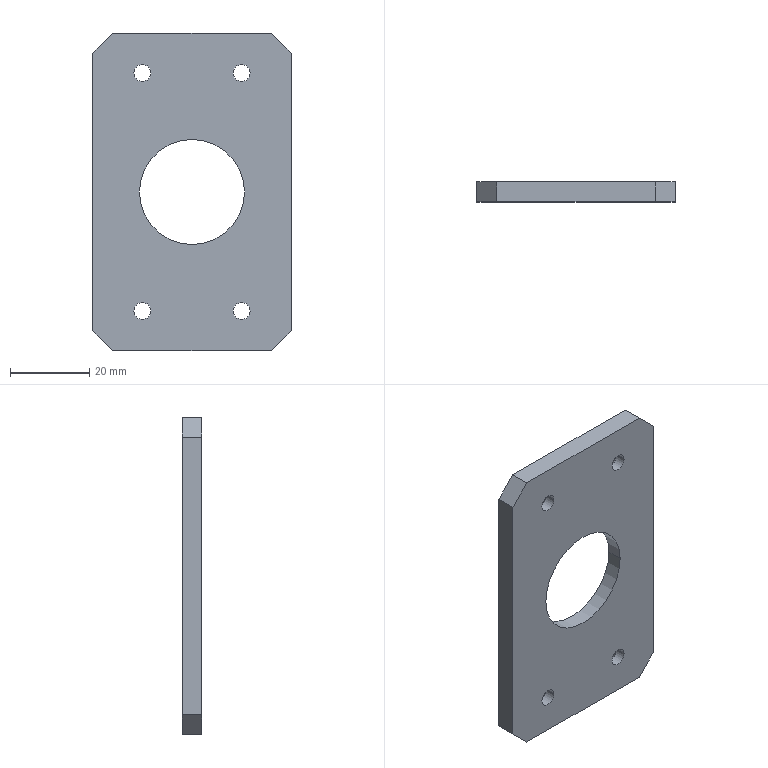Component | SolidWorks | AdjustmentCylinderFixingPlate-1 | 1 solid | 37 faces | box 50 x 5.01 x 80 mm | volume 16157 mm3 | plane 15 | cylinder 14 | cone 8 | commonest cylinder face diameters 4.3 x8 4 x4 26.5 x2
build123d program:
from build123d import *

# Parameters (mm, degrees)
SKETCH1_W                                            = 50
SKETCH1_H                                            = 80
BOSS_EXTRUDE1_DEPTH                                  = 5
CHAMFER1_SIZE                                        = 5
SKETCH2_R                                            = 13.25
CUT_EXTRUDE1_DEPTH                                   = 5
SKETCH3_W                                            = 30
SKETCH3_H                                            = 30
CUT_EXTRUDE2_DEPTH                                   = 1
FILLET1_R                                            = 2
COUNTERSUNK_HOLE_FOR_M4_HEXAGON_SOCKET_C_D           = 4.3
COUNTERSUNK_HOLE_FOR_M4_HEXAGON_SOCKET_C_CSINK_D     = 8.96
COUNTERSUNK_HOLE_FOR_M4_HEXAGON_SOCKET_C_CSINK_ANGLE = 90


with BuildPart() as part:
    # Sketch1 → Boss-Extrude1 (new body)
    with BuildSketch(Plane.XY):
        Rectangle(SKETCH1_W, SKETCH1_H)
    extrude(amount=BOSS_EXTRUDE1_DEPTH)

    # Chamfer1
    chamfer1_edges = [part.edges().sort_by_distance(p)[0] for p in [
        (-25, 40, 2.5),
        (25, 40, 2.5),
        (25, -40, 2.5),
        (-25, -40, 2.5),
    ]]
    chamfer(chamfer1_edges, length=CHAMFER1_SIZE)

    # Sketch2 → Cut-Extrude1 (cut)
    with BuildSketch(Plane.XY.offset(5)):
        Circle(SKETCH2_R)
    extrude(amount=-CUT_EXTRUDE1_DEPTH, mode=Mode.SUBTRACT)

    # Sketch3 → Cut-Extrude2 (cut)
    with BuildSketch(Plane.XY.offset(5)):
        Rectangle(SKETCH3_W, SKETCH3_H)
    extrude(amount=-CUT_EXTRUDE2_DEPTH, mode=Mode.SUBTRACT)

    # Fillet1
    fillet1_edges = [part.edges().sort_by_distance(p)[0] for p in [
        (-15, -15, 4.5),
        (-15, 15, 4.5),
        (15, 15, 4.5),
        (15, -15, 4.5),
    ]]
    fillet(fillet1_edges, radius=FILLET1_R)

    # Countersunk hole for M4 Hexagon Socket C (through all)
    with Locations(Plane.XY.offset(5)):
        with Locations((-12.5, 30), (12.5, 30), (-12.5, -30), (12.5, -30)):
            CounterSinkHole(COUNTERSUNK_HOLE_FOR_M4_HEXAGON_SOCKET_C_D / 2, COUNTERSUNK_HOLE_FOR_M4_HEXAGON_SOCKET_C_CSINK_D / 2, counter_sink_angle=COUNTERSUNK_HOLE_FOR_M4_HEXAGON_SOCKET_C_CSINK_ANGLE)


solid = part.part

# Placed as in the assembly
solid = solid.moved(Location((1702.142, 3968.72, 1079.241), (-90, 0, 0)))